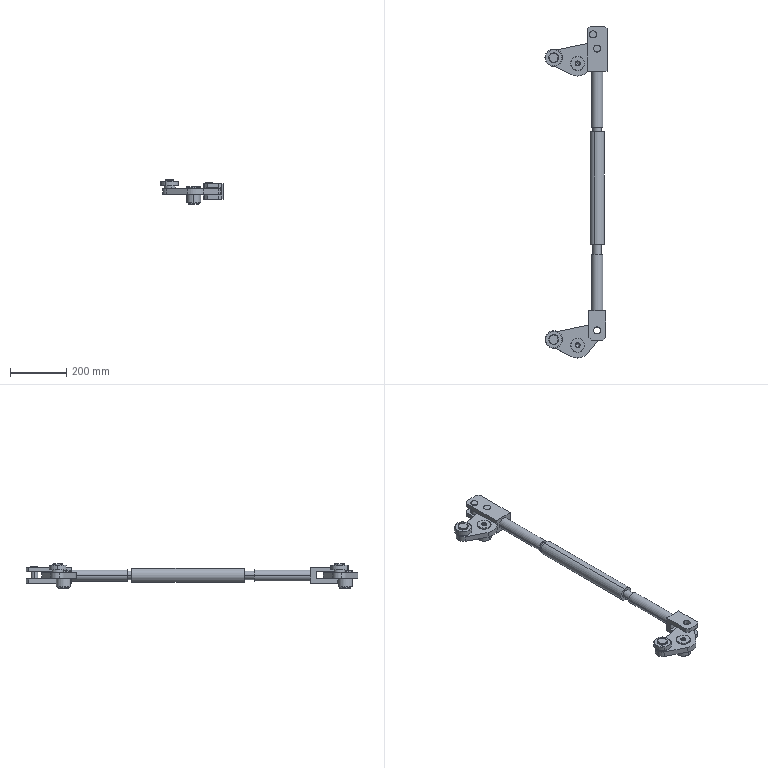Assembly | SolidWorks | mm | 15 component files | 17 solids | 272 faces | box 220.08 x 1177.79 x 86 mm | volume 2748036 mm3 | cylinder 122 | plane 94 | cone 56 | commonest cylinder face diameters 25 x20 30 x20 50 x16 40 x12 35 x12 45 x8 18 x8 20 x8
Bill of materials:
6206Bearing1 | 2 | AISI 1045 Steel, Cold Drawn | Thick flat annular ring (washer-like) with a central through bore; a thin line close to the outer and inner edges of the top face suggests small edge breaks.
AdjustingTieRod1 | 1 | N/A | Long straight round tube of constant outer diameter with a concentric bore and flat square-cut ends.
Axis | 1 |  | Plain solid round cylinder (rod or pin blank) with flat ends, length about 2.4 times diameter.
FixedAxis1 | 2 | N/A | Stepped cylindrical turned body: chamfered top flange, a narrow groove below it, a reduced-diameter upper section, a larger-diameter lower band, and a short reduced chamfered spigot at the bottom. A small central stepped (counterbored) hole opens on the top face.
Left-handTieRod1 | 1 | N/A | Clevis-style rod end: a rectangular forked head with two parallel tabs, each with one aligned cross hole and chamfered end corners, joined to a round shank that steps down to a smaller diameter toward the free end.
M20Bolt1 | 2 |  | Stepped headed pin: a top head flange with two opposite parallel flats and chamfered edges, a cylindrical body, a short reduced neck or undercut, and a smaller cylindrical shank with a chamfered end.
Pin | 1 |  | Plain solid round cylinder with flat ends, length about 2.2 times diameter.
Right-handTieRod1 | 1 | N/A | Forked rod end with a rectangular clevis head that has two parallel tabs, each with two aligned cross holes and chamfered end corners, on a round shank that steps down to a smaller diameter at the free end.
Spacer30101 | 2 |  | Thin-walled short cylindrical ring (sleeve or spacer-like) with a large bore and small chamfers on the outer edges at both ends.
TriangularCrank1 | 2 | N/A | Flat plate of constant thickness with a rounded triangular outline, two smaller through holes at two rounded corners and one larger through hole near the third corner.
Mates:
1. coincident | FixedAxis1-1 plane at (0, 0, 0) dir (1, 0, 0) | assembly plane at (0, 0, 0) dir (1, 0, 0)
2. distance | FixedAxis1-1 plane at (0, 0, 0) dir (0, 1, 0) | FixedAxis1-2 plane at (0, 1000, 0) dir (0, 1, 0)
3. coincident | FixedAxis1-1 plane at (0, 0, 0) dir (0, 0, 1) | FixedAxis1-2 plane at (0, 1000, 0) dir (0, 0, 1)
4. parallel | TriangularCrank1-1 face at (-159.631, 30.137, 27) dir (-0.206, 0.9786, 0) | TriangularCrank1-2 face at (-159.631, 1030.137, 27) dir (-0.206, 0.9786, 0)
5. coincident | TriangularCrank1-1 face at (-12.847, 61.034, 27) dir (0, 0, 1) | TriangularCrank1-2 face at (-12.847, 1061.034, 27) dir (0, 0, 1)
6. concentric | FixedAxis1-1 face at (0, 0, 28) dir (0, 0, 1) r 22.5 | TriangularCrank1-1 face at (0, 0, 7) dir (0, 0, 1) r 22.5
7. distance | FixedAxis1-1 face at (0, 25, 6) dir (0, 0, 1) | TriangularCrank1-1 face at (-12.847, 61.034, 7) dir (0, 0, -1)
8. concentric | FixedAxis1-2 face at (0, 1000, 28) dir (0, 0, 1) r 22.5 | TriangularCrank1-2 face at (0, 1000, 7) dir (0, 0, 1) r 22.5
9. coincident | FixedAxis1-1 plane at (0, 0, 0) dir (1, 0, 0) | FixedAxis1-2 plane at (0, 1000, 0) dir (1, 0, 0)
10. concentric | TriangularCrank1-2 face at (-84.74, 1020.354, 27) dir (0, 0, 1) r 10 | 6206Bearing1-1 face at (-84.74, 1020.354, 20.734) dir (0, 0, -1) r 15
11. coincident | 6206Bearing1-1 face at (-84.74, 1035.354, 53) dir (0, 0, 1) | 6206Bearing1-2 face at (-59.89, 6.4, 53) dir (0, 0, 1)
12. concentric | TriangularCrank1-1 face at (-84.74, 20.354, 27) dir (0, 0, 1) r 10 | 6206Bearing1-2 face at (-84.74, 20.354, 20.734) dir (0, 0, -1) r 15
13. coincident | TriangularCrank1-2 face at (-12.847, 1061.034, 27) dir (0, 0, 1) | M20Bolt1-1 face at (-84.74, 1029.354, 27) dir (0, 0, -1)
14. concentric | TriangularCrank1-2 face at (-84.74, 1020.354, 27) dir (0, 0, 1) r 10 | M20Bolt1-1 face at (-84.74, 1020.354, 58) dir (0, 0, 1) r 10
15. coincident | 6206Bearing1-1 face at (-84.74, 1035.354, 53) dir (0, 0, 1) | M20Bolt1-1 face at (-84.74, 1035.354, 53) dir (0, 0, -1)
16. concentric | 6206Bearing1-1 face at (-84.74, 1020.354, 20.734) dir (0, 0, -1) r 31 | Spacer30101-1 face at (-84.74, 1020.354, 37) dir (0, 0, -1) r 15
17. coincident | TriangularCrank1-2 face at (-12.847, 1061.034, 27) dir (0, 0, 1) | Spacer30101-1 face at (-84.74, 1020.354, 27) dir (0, 0, -1)
18. concentric | M20Bolt1-2 face at (-84.74, 20.354, 58) dir (0, 0, 1) r 15 | Spacer30101-2 face at (-84.74, 20.354, 27) dir (0, 0, 1) r 20
19. coincident | M20Bolt1-1 face at (-84.74, 1037.854, 58) dir (0, 0, 1) | M20Bolt1-2 face at (-84.74, 37.854, 58) dir (0, 0, 1)
20. coincident | M20Bolt1-2 face at (-84.74, 29.354, 27) dir (0, 0, -1) | Spacer30101-2 face at (-84.74, 20.354, 27) dir (0, 0, -1)
21. concentric | 6206Bearing1-2 face at (-84.74, 20.354, 20.734) dir (0, 0, -1) r 15 | M20Bolt1-2 face at (-84.74, 20.354, 58) dir (0, 0, 1) r 10
22. distance | TriangularCrank1-1 face at (-12.847, 61.034, 27) dir (0, 0, 1) | Left-handTieRod1-1 face at (99.344, 102.787, 29.5) dir (0, 0, -1)
23. concentric | TriangularCrank1-1 face at (69.344, 52.787, 7) dir (0, 0, 1) r 12.5 | Left-handTieRod1-1 face at (69.344, 52.787, -15.5) dir (0, 0, 1) r 12.5
24. concentric | AdjustingTieRod1-1 face at (69.344, 757.787, 17) dir (0, -1, 0) r 25 | Left-handTieRod1-1 face at (69.344, 422.787, 17) dir (0, -1, 0) r 20
25. concentric | TriangularCrank1-2 face at (69.344, 1052.787, 7) dir (0, 0, 1) r 12.5 | Right-handTieRod1-1 face at (69.344, 1052.787, 49.5) dir (0, 0, -1) r 12.5
26. coincident | Right-handTieRod1-1 face at (104.344, 972.787, 44.5) dir (0, 0, 1) | Left-handTieRod1-1 face at (99.344, 122.787, 44.5) dir (0, 0, 1)
27. concentric | AdjustingTieRod1-1 face at (69.344, 757.787, 17) dir (0, -1, 0) r 25 | Right-handTieRod1-1 face at (69.344, 672.787, 17) dir (0, 1, 0) r 20
28. distance | Left-handTieRod1-1 face at (69.344, 422.787, 17) dir (0, 1, 0) | AdjustingTieRod1-1 face at (69.344, 357.787, 17) dir (0, -1, 0)
29. parallel | 6206Bearing1-1 plane at (-84.74, 1020.354, 45) dir (1, 0, 0) | assembly plane at (0, 0, 0) dir (1, 0, 0)
30. concentric | Right-handTieRod1-1 face at (69.344, 1052.787, 49.5) dir (0, 0, -1) r 12.5 | Pin-1 face at (69.344, 1052.787, 44.5) dir (0, 0, -1) r 12.5
31. coincident | Right-handTieRod1-1 face at (104.344, 972.787, 44.5) dir (0, 0, 1) | Pin-1 face at (69.344, 1052.787, 44.5) dir (0, 0, 1)
32. concentric | Right-handTieRod1-1 face at (54.344, 1102.787, 49.5) dir (0, 0, -1) r 12.5 | Axis-1 face at (54.344, 1102.787, 47) dir (0, 0, -1) r 12.5
33. distance | Axis-1 face at (54.344, 1102.787, 47) dir (0, 0, 1) | Right-handTieRod1-1 face at (104.344, 972.787, 44.5) dir (0, 0, 1)